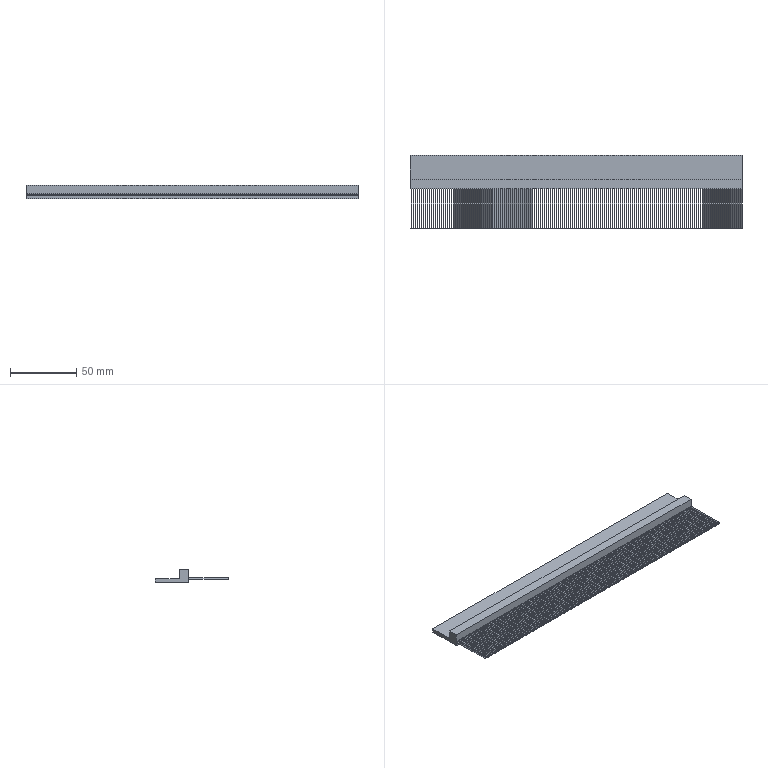Component | SolidWorks | Brush-1 | 1 solid | 508 faces | box 250 x 55 x 10 mm | volume 34923 mm3 | cylinder 333 | plane 175 | commonest cylinder face diameters 1 x333
build123d program:
from build123d import *

# Parameters (mm, degrees)
BOSS_EXTRUDE1_DEPTH = 125
SWEEP1_PROFILE_R    = 0.5
LPATTERN1_COUNT     = 167
LPATTERN1_PITCH     = 1.5
SKETCH171_W         = 100
SKETCH171_H         = 100
CUT_EXTRUDE2_DEPTH  = 252.992


with BuildPart() as part:
    # Sketch1 → Boss-Extrude1 (new, symmetric)
    with BuildSketch(Plane.XY):
        Polygon((0, 0), (0, 25), (3, 25), (3, 7), (10, 7), (10, 0), align=None)
    extrude(amount=BOSS_EXTRUDE1_DEPTH, both=True)

    # Sweep1: sweep along a path in Sketch3
    with BuildLine(Plane(origin=(3, 0, 0), x_dir=(0, 0, -1), z_dir=(1, 0, 0))) as sweep1_path:
        Line((125, 0), (125, -30))
    # Sweep1 profile (on start of the path) → Sweep1 (sweep)
    with BuildSketch(Plane(origin=(3, 0, -125), x_dir=(-1, 0, 0), z_dir=(0, -1, 0))):
        Circle(SWEEP1_PROFILE_R)
    sweep1 = sweep(path=sweep1_path.line)

    # LPattern1: Sweep1 ×167
    with Locations(*[(0, 0, i * LPATTERN1_PITCH) for i in range(1, LPATTERN1_COUNT)]):
        add(sweep1)

    # Sketch171 → Cut-Extrude2 (cut, through all)
    with BuildSketch(Plane(origin=(0, 0, -125), x_dir=(-1, 0, 0), z_dir=(0, 0, -1))):
        Rectangle(SKETCH171_W, SKETCH171_H)
    extrude(amount=CUT_EXTRUDE2_DEPTH, mode=Mode.SUBTRACT)


solid = part.part

# Placed as in the assembly
solid = solid.moved(Location((173.5, 270, 125), (0, -90, 0)))